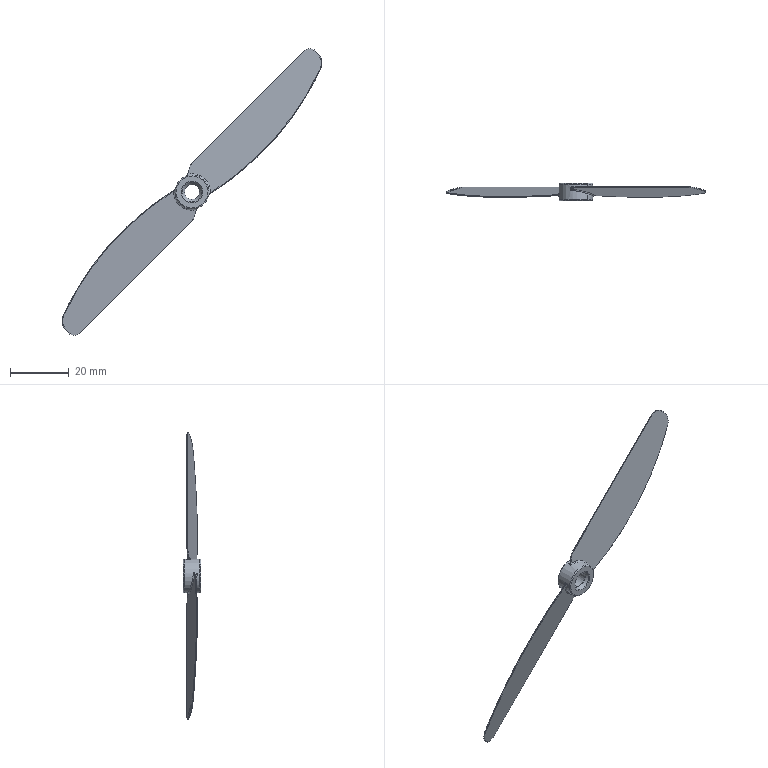Component | SolidWorks | 9.P-1 | 1 solid | 102 faces | box 88.15 x 6 x 97.34 mm | volume 933 mm3 | spline 30 | torus 24 | cylinder 22 | plane 22 | cone 4 | commonest cylinder face diameters 0.2 x12 10 x4 5 x2 11.5 x2 6 x2